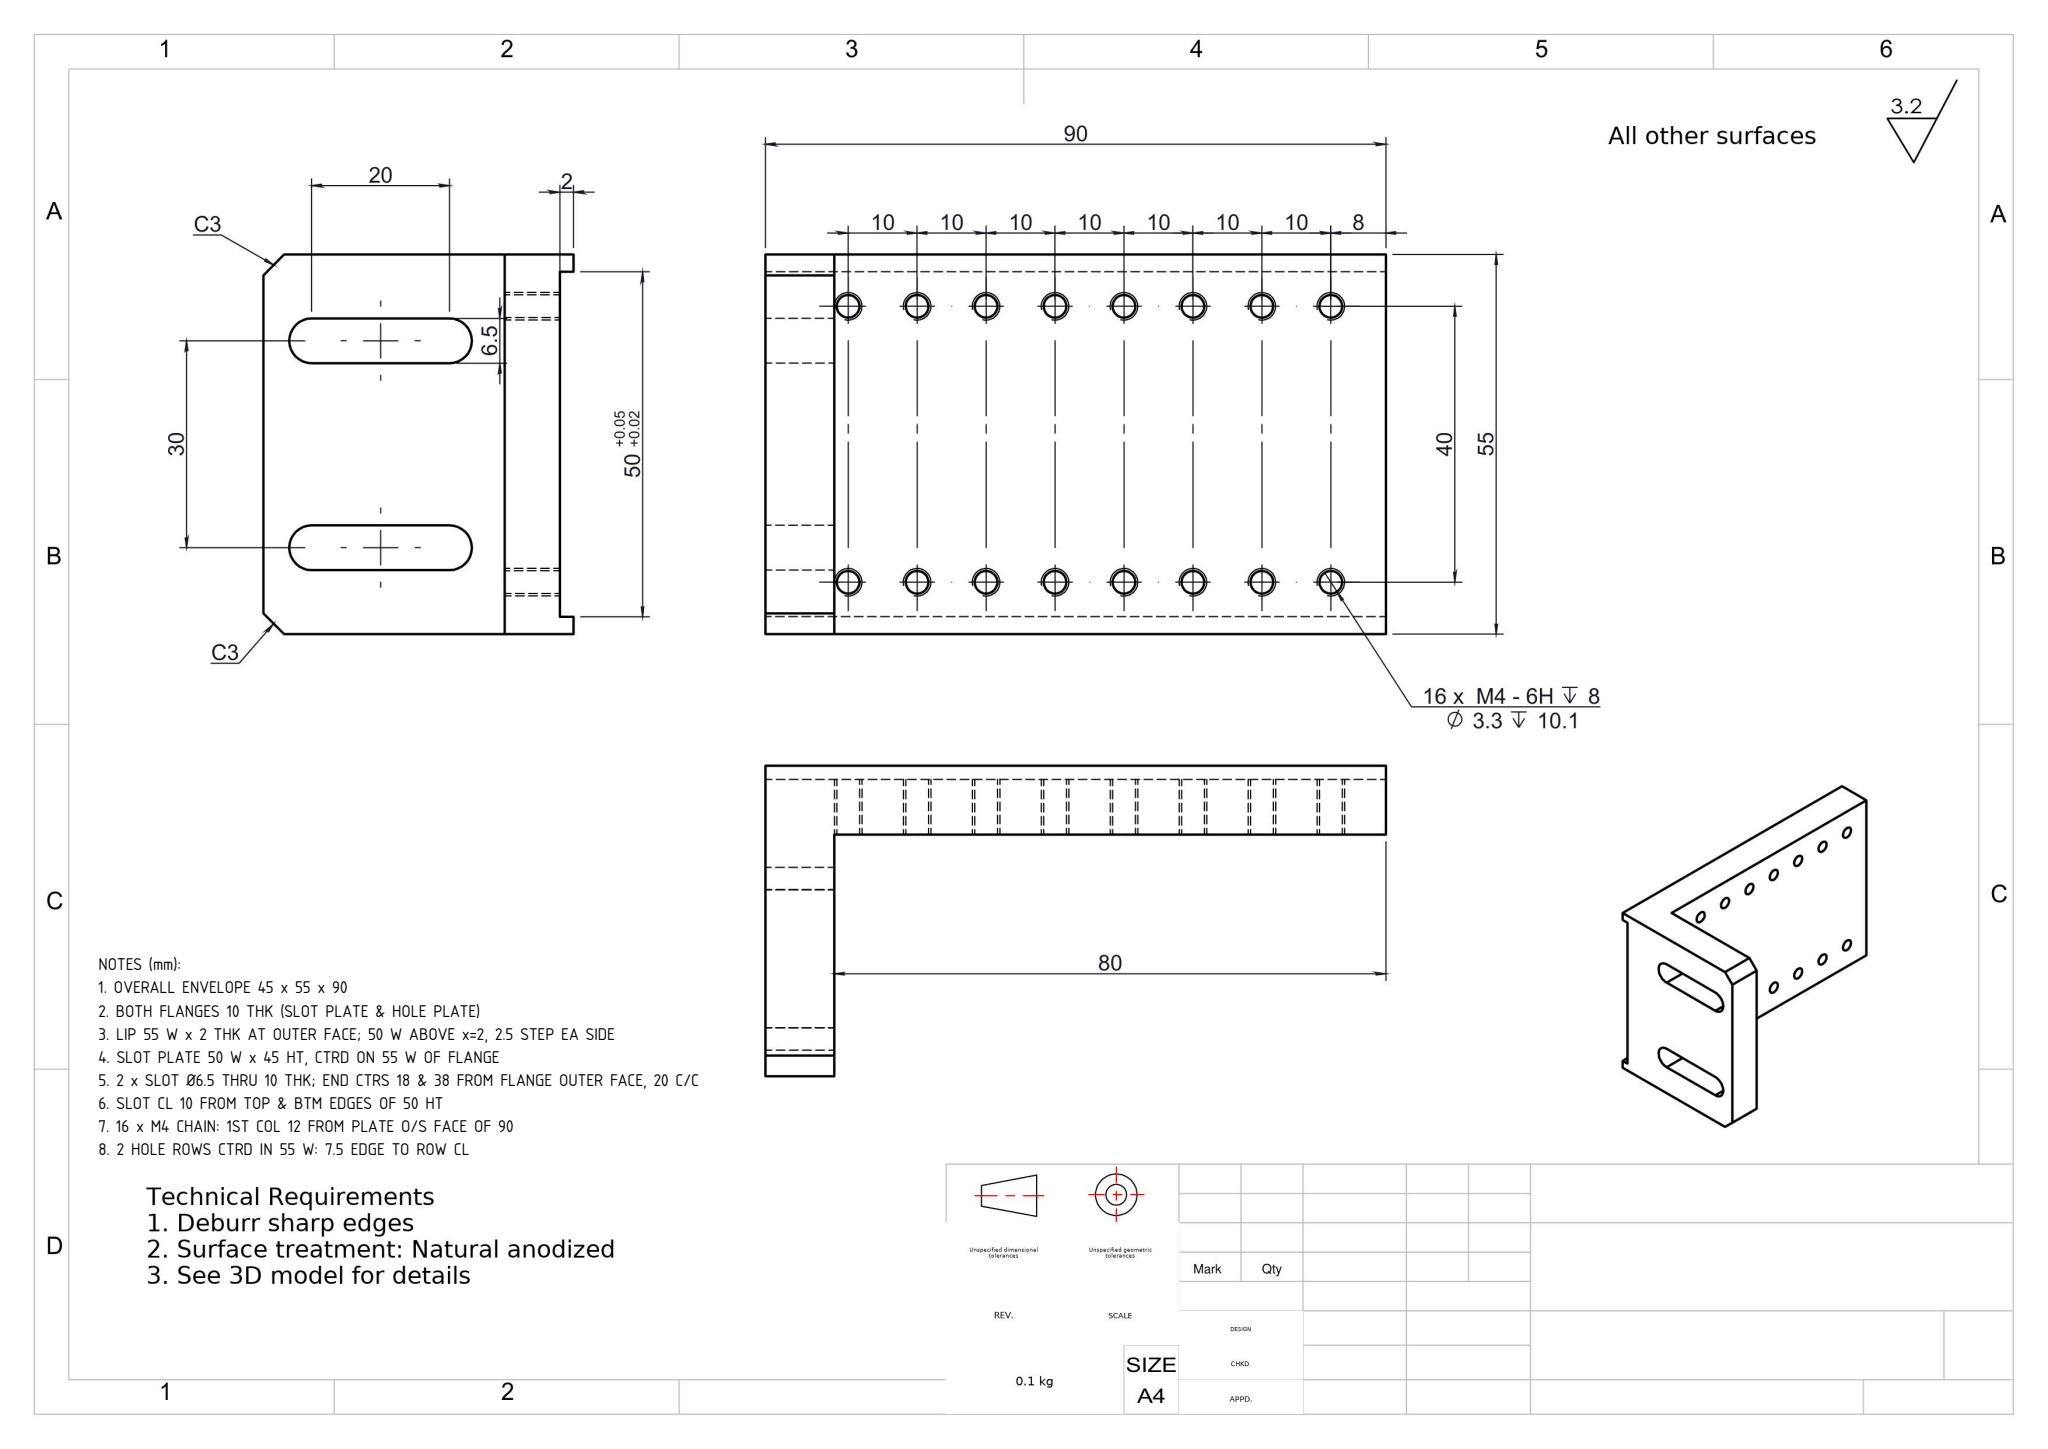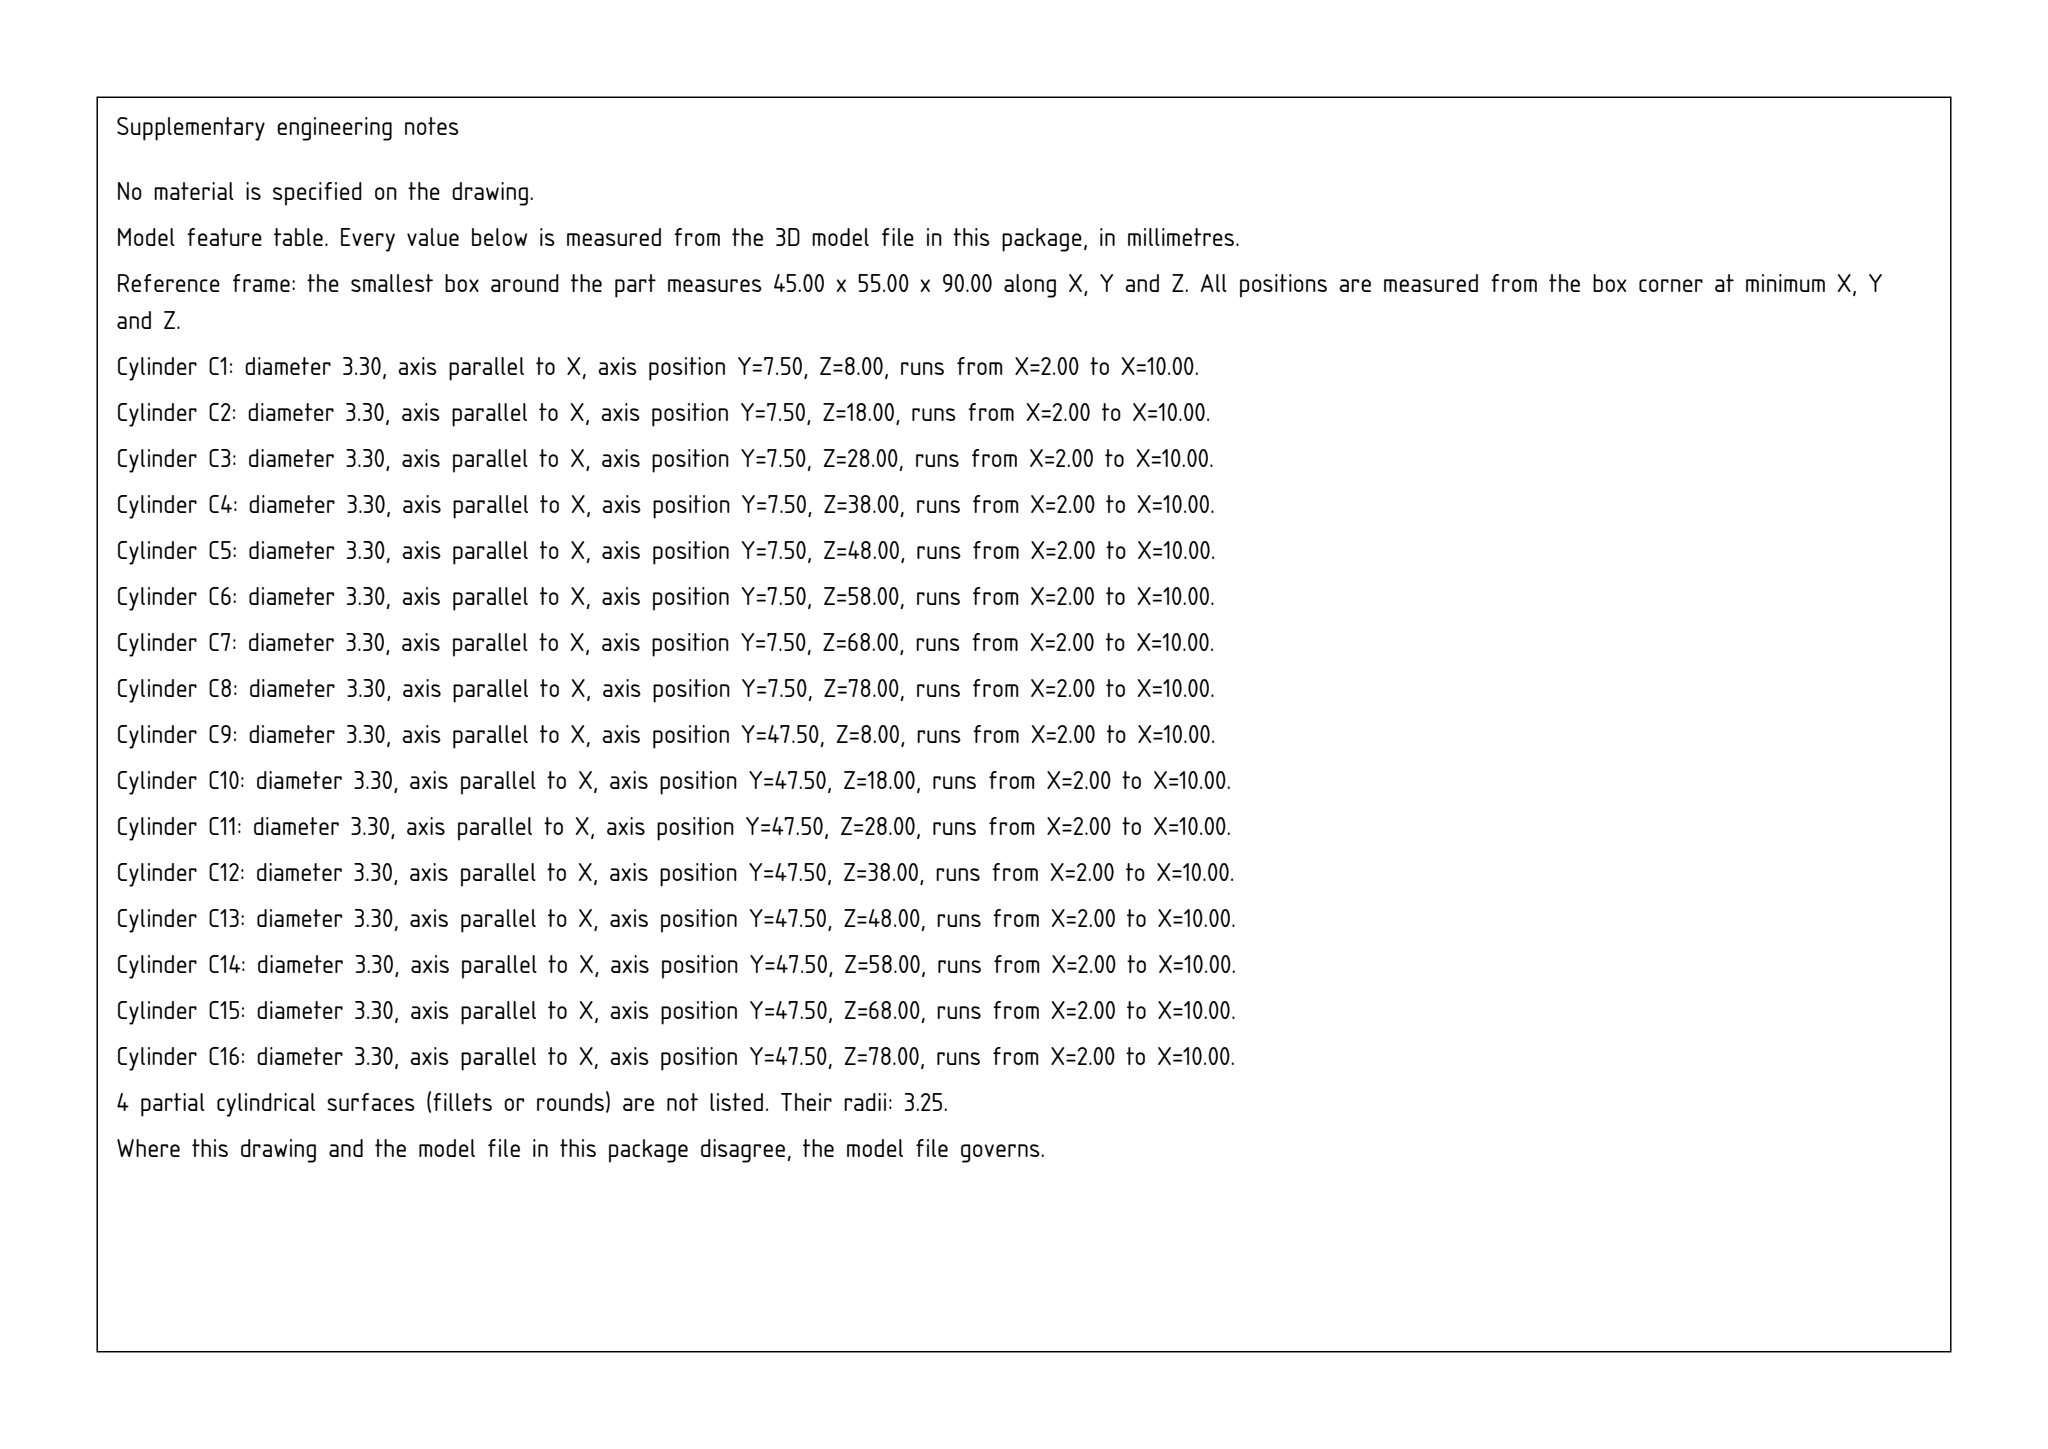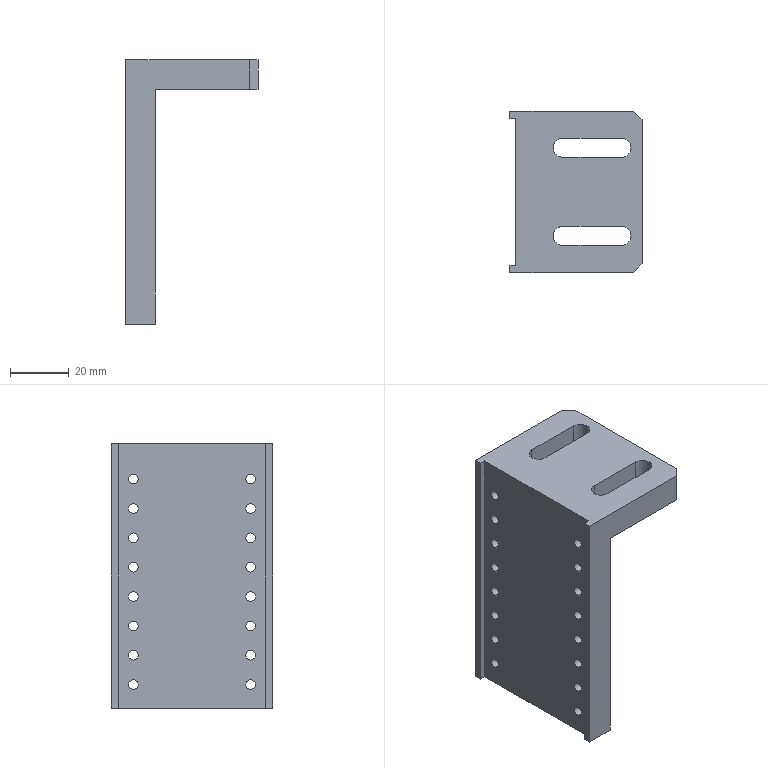Part | SolidWorks | mm | 1 solid | 56 faces | box 45 x 55 x 90 mm | volume 55302 mm3 | cylinder 38 | plane 18 | commonest cylinder face diameters 3.3 x32 6.5 x6
Drawing notes:
OVERALL ENVELOPE 45 x 55 x 90 | from the solid: bbox_xyz [45.0, 55.0, 90.0]
BOTH FLANGES 10 THK (SLOT PLATE & HOLE PLATE) | from the solid: x-planes 0 & 10 (horiz flange); z-planes 80 & 90 (vert plate) -> 10 wall each
LIP 55 W x 2 THK AT OUTER FACE; 50 W ABOVE x=2, 2.5 STEP EA SIDE | from the solid: y-planes 0/55 and 2.5/52.5 with x-plane 2.0; 50 +0.05/+0.02 width above x=2
SLOT PLATE 50 W x 45 HT, CTRD ON 55 W OF FLANGE | from the solid: plate y 2.5-52.5 in bbox y=55; plate x 0-45
2 x SLOT Ø6.5 THRU 10 THK; END CTRS 18 & 38 FROM FLANGE OUTER FACE, 20 C/C | from the solid: Ø6.5 slot-end cyls axis z, len 10, at x=18 and x=38; flange outer face x=0
SLOT CL 10 FROM TOP & BTM EDGES OF 50 HT | from the solid: slot cyls y=12.5 & 42.5; plate edges y=2.5 & 52.5
16 x M4 CHAIN: 1ST COL 12 FROM PLATE O/S FACE OF 90 | from the solid: hole z=78 nearest z=90 face; cols z=8..78 step 10, 8 from z=0 end
2 HOLE ROWS CTRD IN 55 W: 7.5 EDGE TO ROW CL | from the solid: hole rows y=7.5 and y=47.5 in 55 width (40 apart, centered)